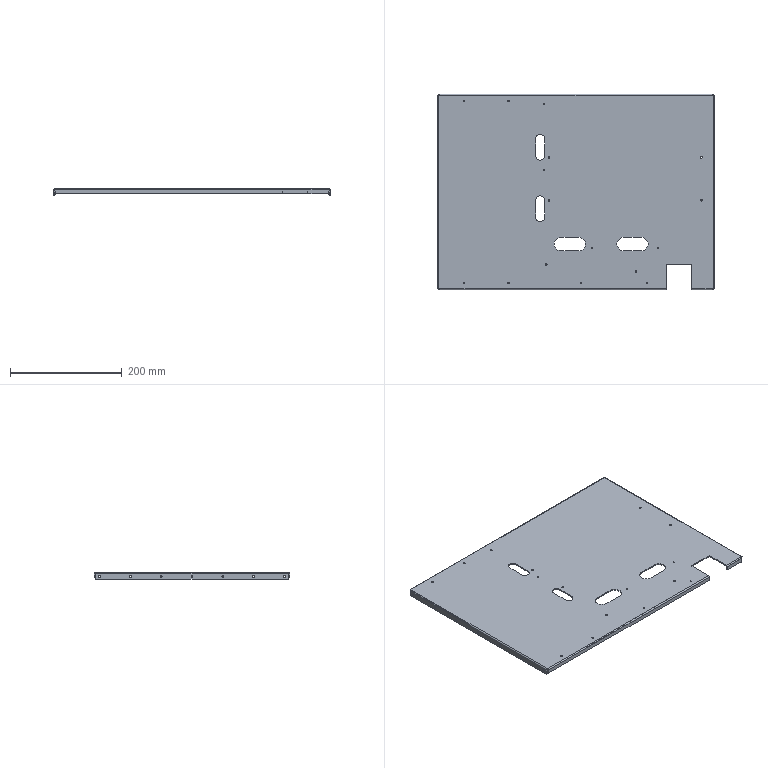CAM job | Mastercam | mm | 4 operations | part box 493.8 x 350 x 12
1. Contour (Ramp) | 10 - 10 平铣刀
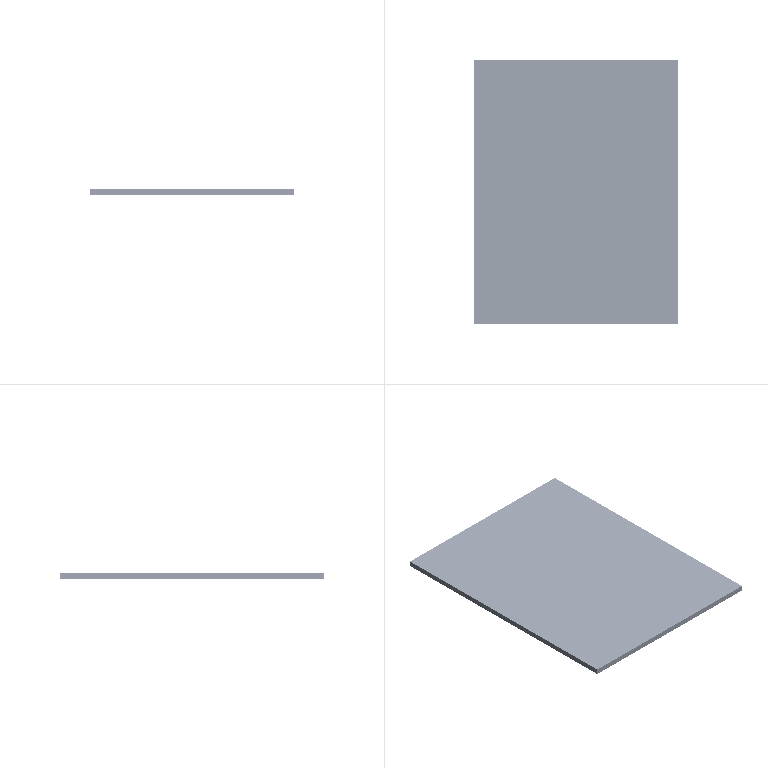2. Contour (Remachining) | 2 - 2 平铣刀
3. Contour (2D) | 10 - 10 平铣刀
4. Drill/Counterbore | 7 - 4 倒角刀